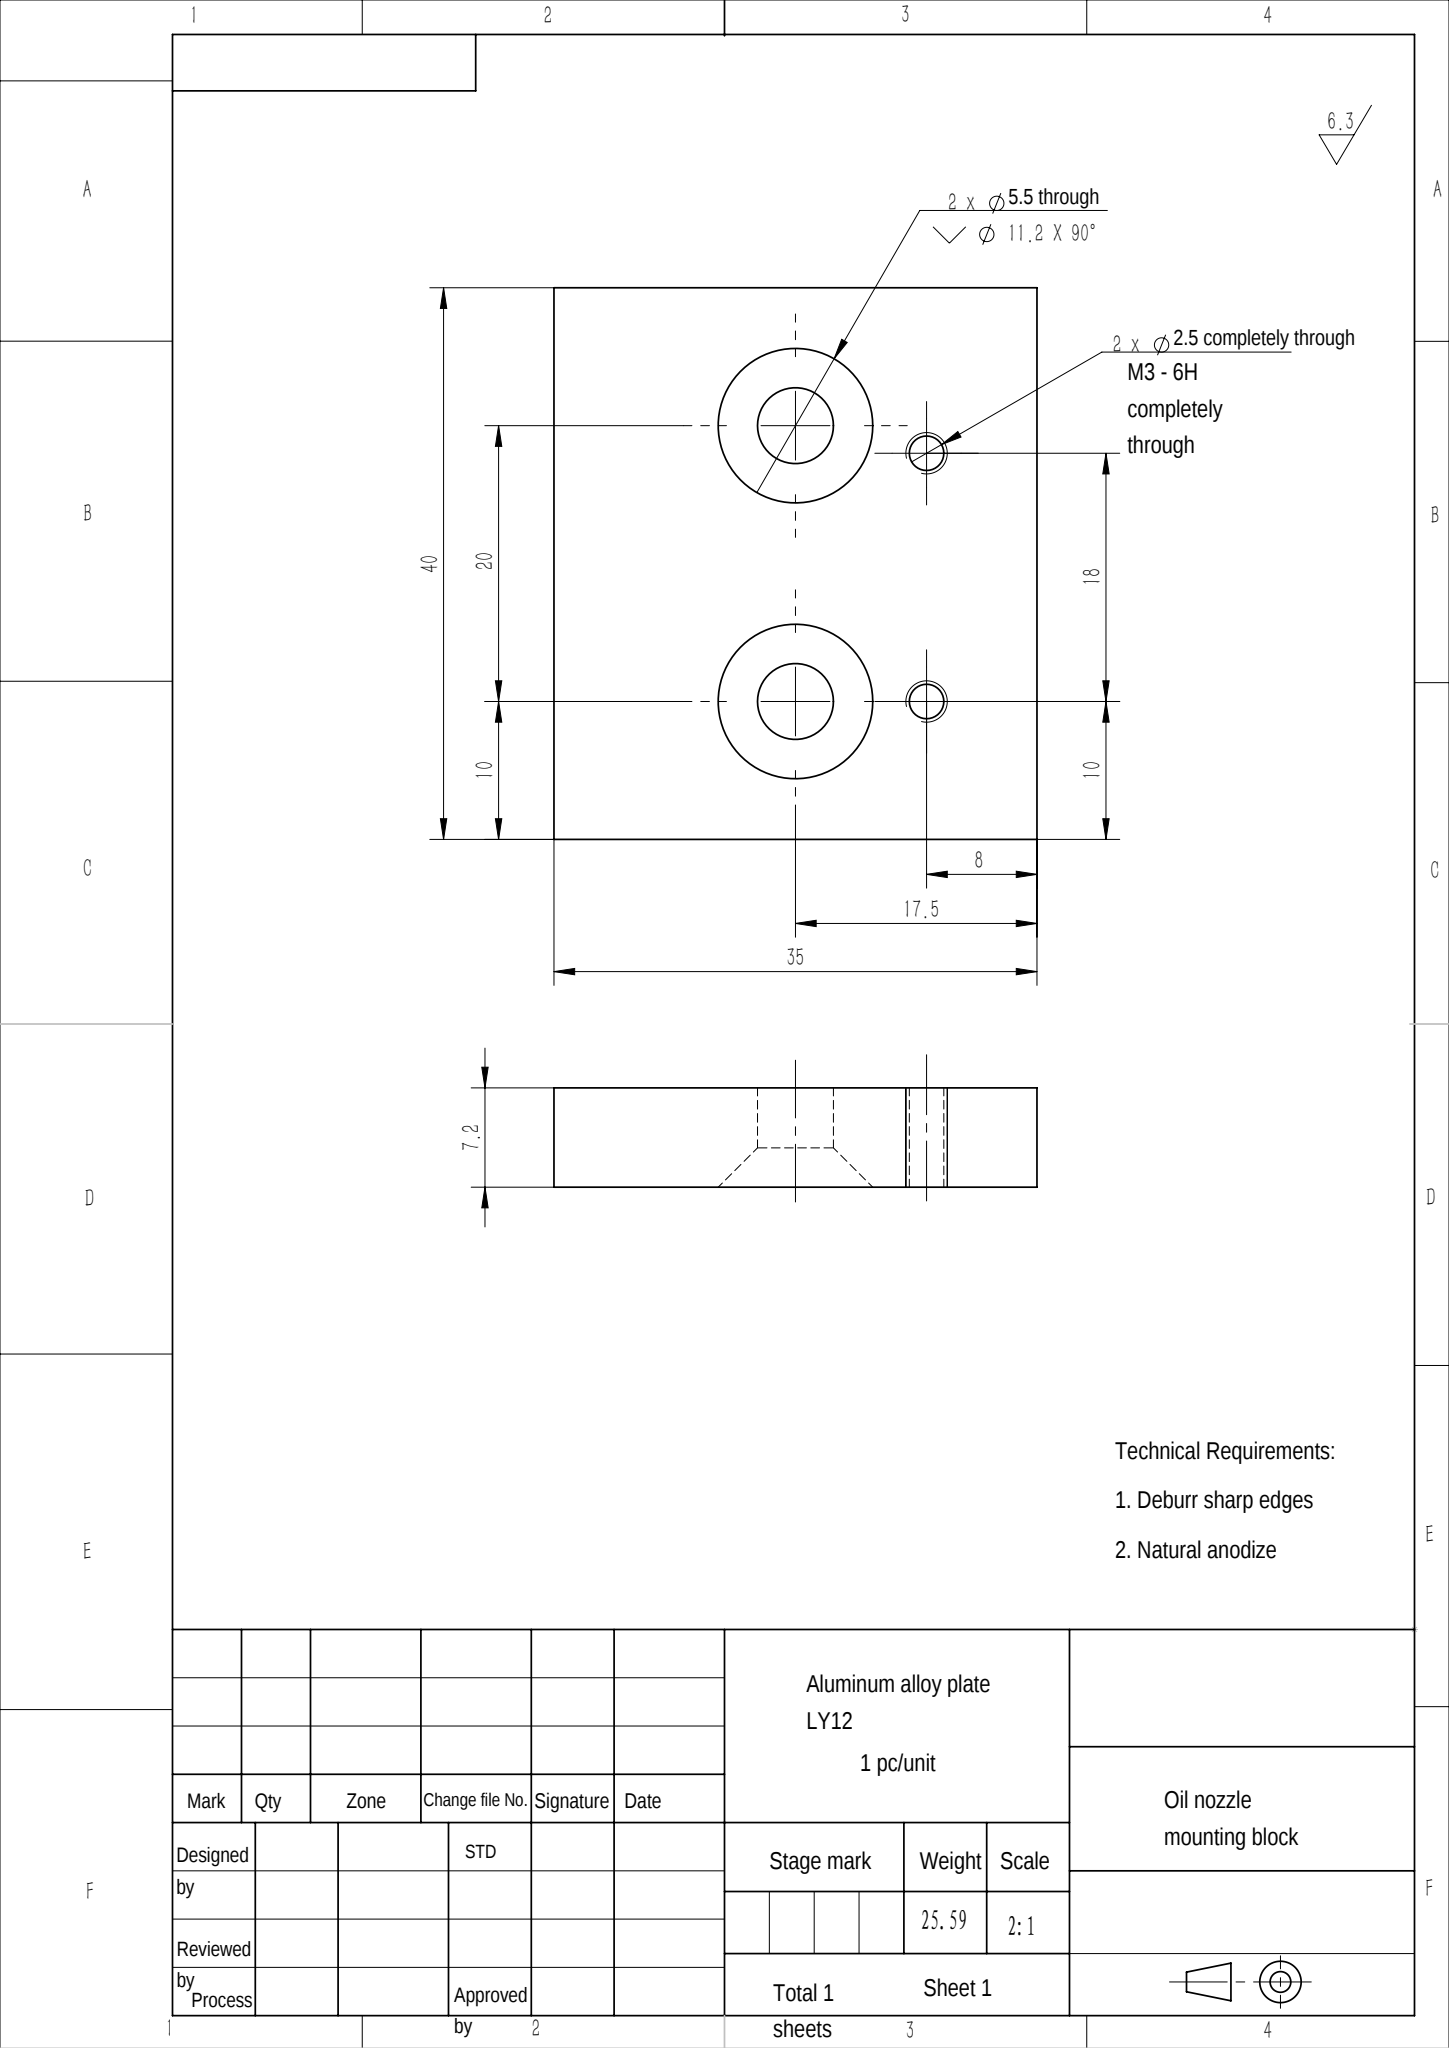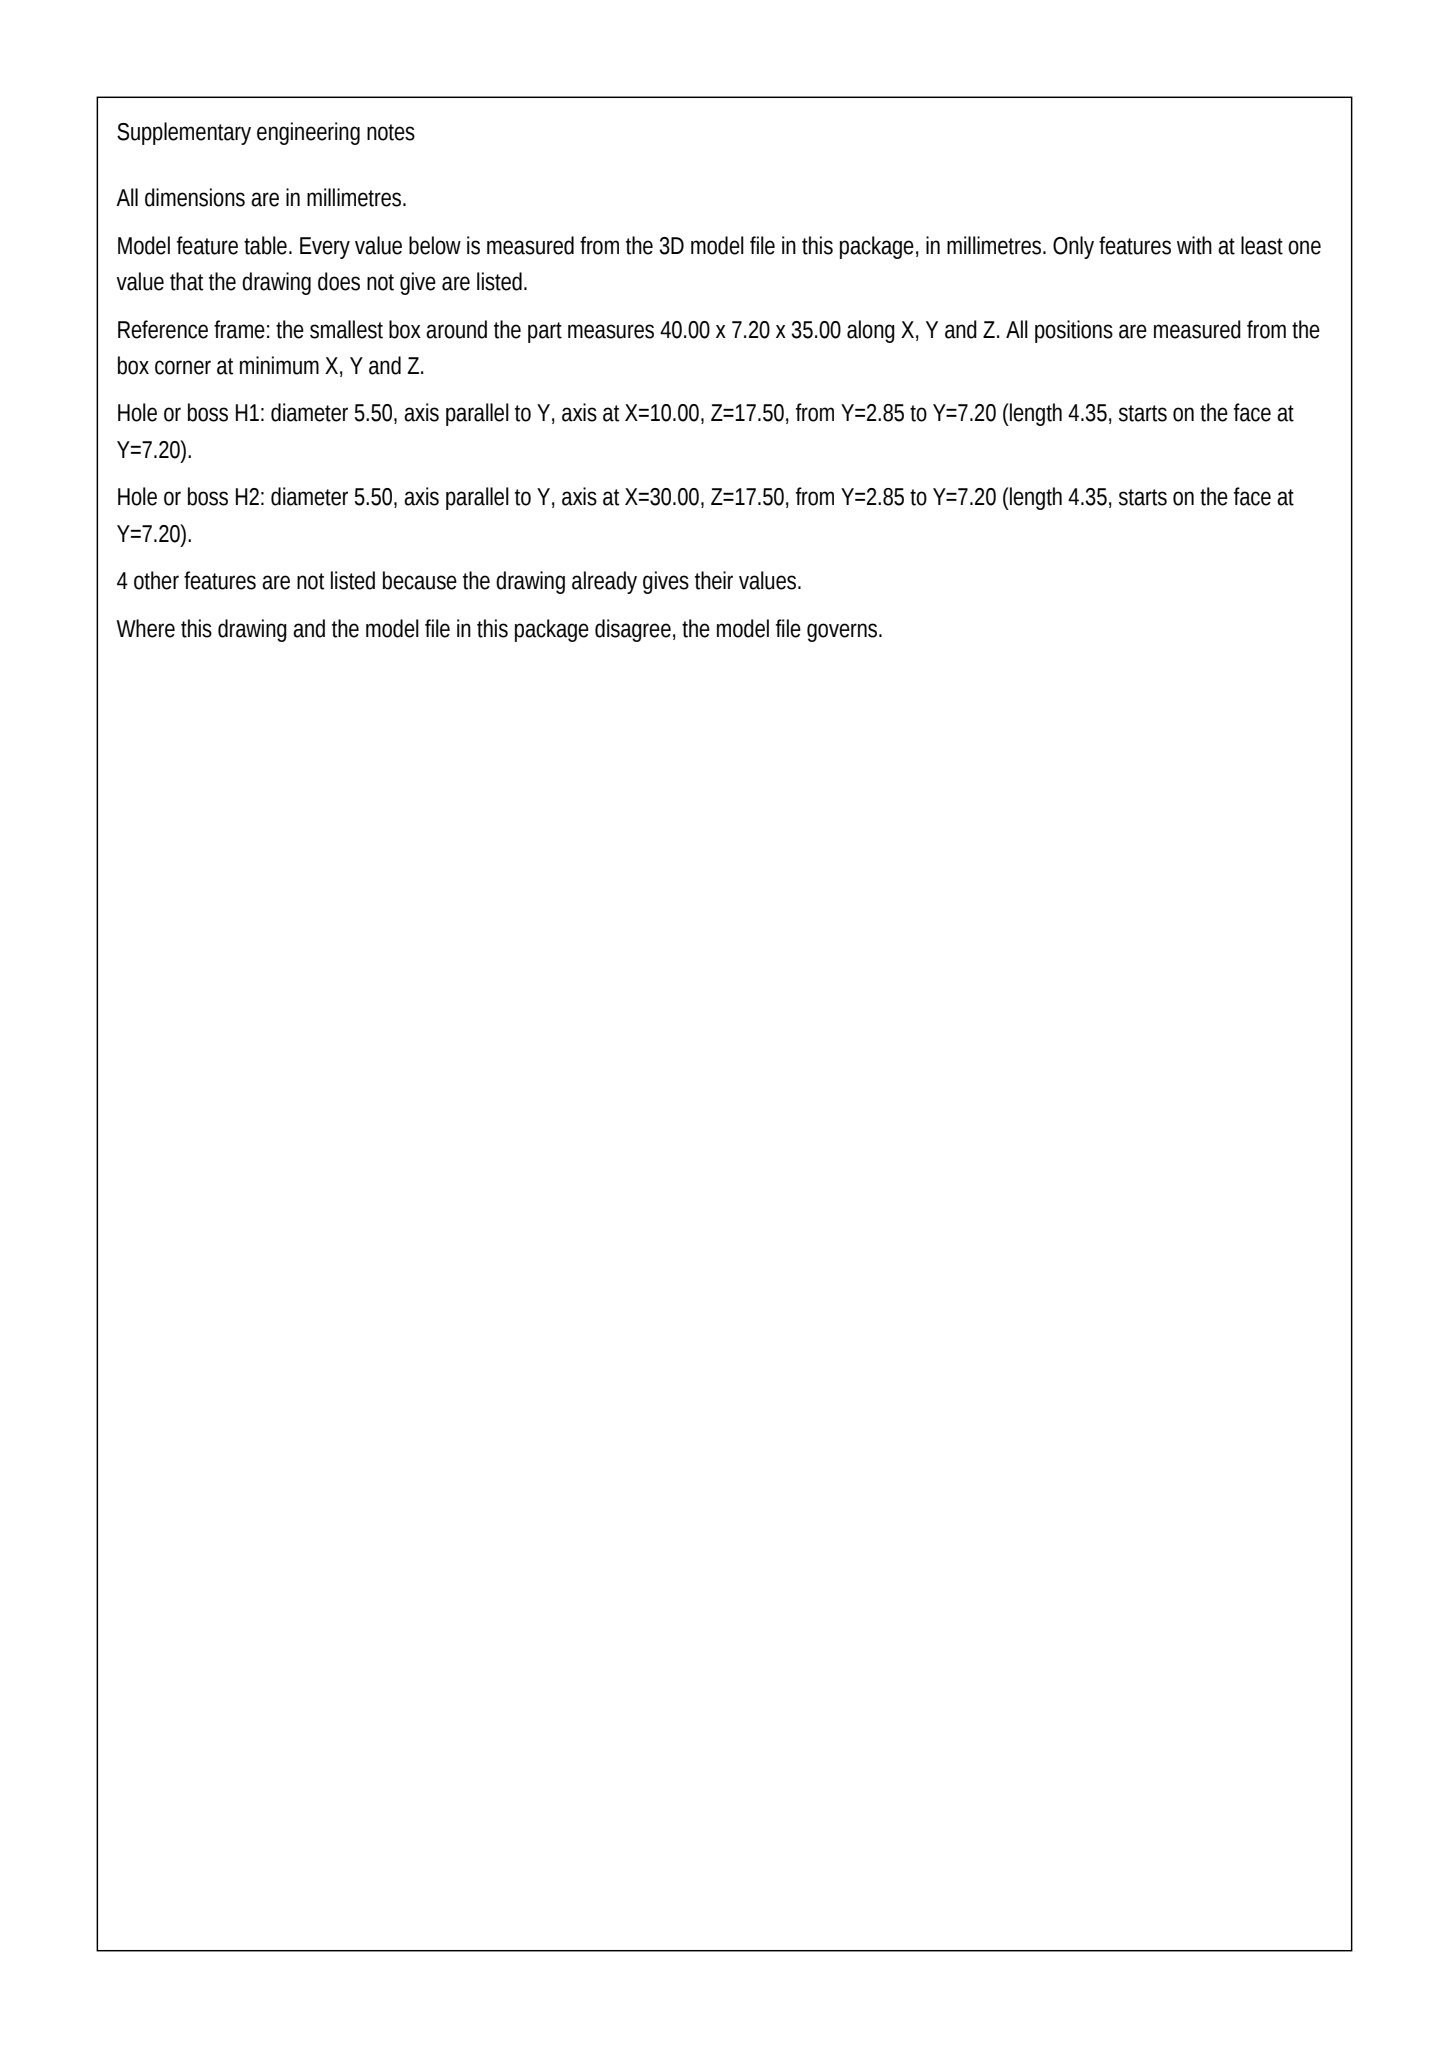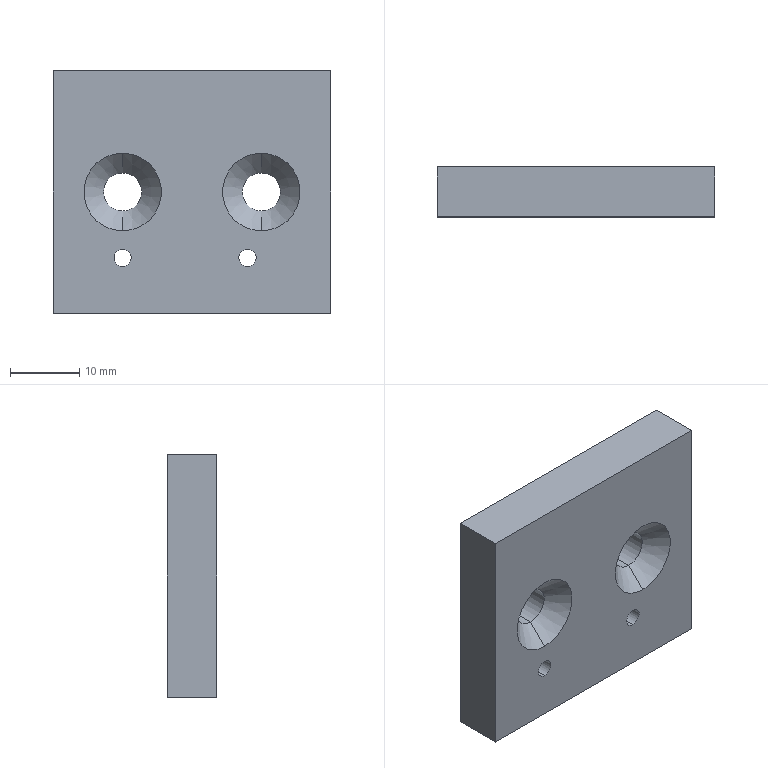Part | SolidWorks | mm | material Aluminum alloy plate LY12 | 1 solid | 18 faces | box 40 x 7.2 x 35 mm | volume 9478 mm3 | cylinder 8 | plane 6 | cone 4 | commonest cylinder face diameters 5.5 x4 2.5 x4
build123d program:
from build123d import *

# Parameters (mm, degrees)
SKETCH1_W                                           = 40
SKETCH1_H                                           = 35
BOSS_EXTRUDE1_DEPTH                                 = 7.2
M3_TAPPED_HOLE1_D                                   = 2.5
TAPERED_COUNTERSUNK_HOLE_FOR_M5_HEXAGON_D           = 5.5
TAPERED_COUNTERSUNK_HOLE_FOR_M5_HEXAGON_CSINK_D     = 11.2
TAPERED_COUNTERSUNK_HOLE_FOR_M5_HEXAGON_CSINK_ANGLE = 90


with BuildPart() as part:
    # Sketch1 → Boss-Extrude1 (new body)
    with BuildSketch(Plane(origin=(0, 0, 0), x_dir=(1, 0, 0), z_dir=(0, 1, 0))):
        Rectangle(SKETCH1_W, SKETCH1_H)
    extrude(amount=BOSS_EXTRUDE1_DEPTH)

    # M3 Tapped Hole1 (through all)
    with Locations(Plane(origin=(0, 0, 0), x_dir=(-1, 0, 0), z_dir=(0, -1, 0))):
        with Locations((10, 9.5), (-8, 9.5)):
            Hole(M3_TAPPED_HOLE1_D / 2)

    # Tapered Countersunk Hole for M5 Hexagon (through all)
    with Locations(Plane(origin=(0, 0, 0), x_dir=(-1, 0, 0), z_dir=(0, -1, 0))):
        with Locations((-10, 0), (10, 0)):
            CounterSinkHole(TAPERED_COUNTERSUNK_HOLE_FOR_M5_HEXAGON_D / 2, TAPERED_COUNTERSUNK_HOLE_FOR_M5_HEXAGON_CSINK_D / 2, counter_sink_angle=TAPERED_COUNTERSUNK_HOLE_FOR_M5_HEXAGON_CSINK_ANGLE)


solid = part.part
STEP:
#1=CARTESIAN_POINT('',(10.,2.85,2.75));
#2=VERTEX_POINT('',#1);
#3=CARTESIAN_POINT('',(10.,2.85,-2.75));
#4=VERTEX_POINT('',#3);
#5=CARTESIAN_POINT('',(10.,2.85,-0.));
#6=DIRECTION('',(0.,-1.,0.));
#7=DIRECTION('',(0.,0.,-1.));
#8=AXIS2_PLACEMENT_3D('',#5,#6,#7);
#9=CIRCLE('',#8,2.75);
#10=EDGE_CURVE('',#2,#4,#9,.T.);
#11=ORIENTED_EDGE('',*,*,#10,.F.);
#12=CARTESIAN_POINT('',(10.,-0.,5.6));
#13=VERTEX_POINT('',#12);
#14=CARTESIAN_POINT('',(10.,-0.,5.6));
#15=DIRECTION('',(0.,-0.7071,0.7071));
#16=VECTOR('',#15,1000.);
#17=LINE('',#14,#16);
#18=EDGE_CURVE('',#2,#13,#17,.T.);
#19=ORIENTED_EDGE('',*,*,#18,.T.);
#20=CARTESIAN_POINT('',(10.,-0.,-5.6));
#21=VERTEX_POINT('',#20);
#22=CARTESIAN_POINT('',(10.,-0.,-0.));
#23=DIRECTION('',(0.,-1.,0.));
#24=DIRECTION('',(0.,0.,-1.));
#25=AXIS2_PLACEMENT_3D('',#22,#23,#24);
#26=CIRCLE('',#25,5.6);
#27=EDGE_CURVE('',#13,#21,#26,.T.);
#28=ORIENTED_EDGE('',*,*,#27,.T.);
#29=CARTESIAN_POINT('',(10.,-0.,-5.6));
#30=DIRECTION('',(0.,-0.7071,-0.7071));
#31=VECTOR('',#30,1000.);
#32=LINE('',#29,#31);
#33=EDGE_CURVE('',#4,#21,#32,.T.);
#34=ORIENTED_EDGE('',*,*,#33,.F.);
#35=EDGE_LOOP('',(#11,#19,#28,#34));
#36=FACE_OUTER_BOUND('',#35,.T.);
#37=CARTESIAN_POINT('',(10.,-0.,-0.));
#38=DIRECTION('',(0.,-1.,0.));
#39=DIRECTION('',(0.,0.,-1.));
#40=AXIS2_PLACEMENT_3D('',#37,#38,#39);
#41=CONICAL_SURFACE('',#40,5.6,0.7854);
#42=ADVANCED_FACE('',(#36),#41,.F.);
#43=CARTESIAN_POINT('',(10.,7.2,-2.75));
#44=VERTEX_POINT('',#43);
#45=CARTESIAN_POINT('',(10.,7.2,2.75));
#46=VERTEX_POINT('',#45);
#47=CARTESIAN_POINT('',(10.,7.2,-0.));
#48=DIRECTION('',(0.,1.,0.));
#49=DIRECTION('',(0.,0.,1.));
#50=AXIS2_PLACEMENT_3D('',#47,#48,#49);
#51=CIRCLE('',#50,2.75);
#52=EDGE_CURVE('',#44,#46,#51,.T.);
#53=ORIENTED_EDGE('',*,*,#52,.T.);
#54=CARTESIAN_POINT('',(10.,0.,2.75));
#55=DIRECTION('',(0.,-1.,0.));
#56=VECTOR('',#55,1000.);
#57=LINE('',#54,#56);
#58=EDGE_CURVE('',#46,#2,#57,.T.);
#59=ORIENTED_EDGE('',*,*,#58,.T.);
#60=ORIENTED_EDGE('',*,*,#10,.T.);
#61=CARTESIAN_POINT('',(10.,0.,-2.75));
#62=DIRECTION('',(0.,-1.,0.));
#63=VECTOR('',#62,1000.);
#64=LINE('',#61,#63);
#65=EDGE_CURVE('',#44,#4,#64,.T.);
#66=ORIENTED_EDGE('',*,*,#65,.F.);
#67=EDGE_LOOP('',(#53,#59,#60,#66));
#68=FACE_OUTER_BOUND('',#67,.T.);
#69=CARTESIAN_POINT('',(10.,0.,-0.));
#70=DIRECTION('',(0.,-1.,0.));
#71=DIRECTION('',(0.,0.,-1.));
#72=AXIS2_PLACEMENT_3D('',#69,#70,#71);
#73=CYLINDRICAL_SURFACE('',#72,2.75);
#74=ADVANCED_FACE('',(#68),#73,.F.);
#75=CARTESIAN_POINT('',(-10.,2.85,2.75));
#76=VERTEX_POINT('',#75);
#77=CARTESIAN_POINT('',(-10.,2.85,-2.75));
#78=VERTEX_POINT('',#77);
#79=CARTESIAN_POINT('',(-10.,2.85,-0.));
#80=DIRECTION('',(0.,-1.,0.));
#81=DIRECTION('',(0.,0.,-1.));
#82=AXIS2_PLACEMENT_3D('',#79,#80,#81);
#83=CIRCLE('',#82,2.75);
#84=EDGE_CURVE('',#76,#78,#83,.T.);
#85=ORIENTED_EDGE('',*,*,#84,.F.);
#86=CARTESIAN_POINT('',(-10.,-0.,5.6));
#87=VERTEX_POINT('',#86);
#88=CARTESIAN_POINT('',(-10.,-0.,5.6));
#89=DIRECTION('',(0.,-0.7071,0.7071));
#90=VECTOR('',#89,1000.);
#91=LINE('',#88,#90);
#92=EDGE_CURVE('',#76,#87,#91,.T.);
#93=ORIENTED_EDGE('',*,*,#92,.T.);
#94=CARTESIAN_POINT('',(-10.,-0.,-5.6));
#95=VERTEX_POINT('',#94);
#96=CARTESIAN_POINT('',(-10.,-0.,-0.));
#97=DIRECTION('',(0.,-1.,0.));
#98=DIRECTION('',(0.,0.,-1.));
#99=AXIS2_PLACEMENT_3D('',#96,#97,#98);
#100=CIRCLE('',#99,5.6);
#101=EDGE_CURVE('',#87,#95,#100,.T.);
#102=ORIENTED_EDGE('',*,*,#101,.T.);
#103=CARTESIAN_POINT('',(-10.,-0.,-5.6));
#104=DIRECTION('',(0.,-0.7071,-0.7071));
#105=VECTOR('',#104,1000.);
#106=LINE('',#103,#105);
#107=EDGE_CURVE('',#78,#95,#106,.T.);
#108=ORIENTED_EDGE('',*,*,#107,.F.);
#109=EDGE_LOOP('',(#85,#93,#102,#108));
#110=FACE_OUTER_BOUND('',#109,.T.);
#111=CARTESIAN_POINT('',(-10.,-0.,-0.));
#112=DIRECTION('',(0.,-1.,0.));
#113=DIRECTION('',(0.,0.,-1.));
#114=AXIS2_PLACEMENT_3D('',#111,#112,#113);
#115=CONICAL_SURFACE('',#114,5.6,0.7854);
#116=ADVANCED_FACE('',(#110),#115,.F.);
#117=CARTESIAN_POINT('',(-10.,7.2,-2.75));
#118=VERTEX_POINT('',#117);
#119=CARTESIAN_POINT('',(-10.,7.2,2.75));
#120=VERTEX_POINT('',#119);
#121=CARTESIAN_POINT('',(-10.,7.2,-0.));
#122=DIRECTION('',(0.,1.,0.));
#123=DIRECTION('',(0.,0.,1.));
#124=AXIS2_PLACEMENT_3D('',#121,#122,#123);
#125=CIRCLE('',#124,2.75);
#126=EDGE_CURVE('',#118,#120,#125,.T.);
#127=ORIENTED_EDGE('',*,*,#126,.T.);
#128=CARTESIAN_POINT('',(-10.,0.,2.75));
#129=DIRECTION('',(0.,-1.,0.));
#130=VECTOR('',#129,1000.);
#131=LINE('',#128,#130);
#132=EDGE_CURVE('',#120,#76,#131,.T.);
#133=ORIENTED_EDGE('',*,*,#132,.T.);
#134=ORIENTED_EDGE('',*,*,#84,.T.);
#135=CARTESIAN_POINT('',(-10.,0.,-2.75));
#136=DIRECTION('',(0.,-1.,0.));
#137=VECTOR('',#136,1000.);
#138=LINE('',#135,#137);
#139=EDGE_CURVE('',#118,#78,#138,.T.);
#140=ORIENTED_EDGE('',*,*,#139,.F.);
#141=EDGE_LOOP('',(#127,#133,#134,#140));
#142=FACE_OUTER_BOUND('',#141,.T.);
#143=CARTESIAN_POINT('',(-10.,0.,-0.));
#144=DIRECTION('',(0.,-1.,0.));
#145=DIRECTION('',(0.,0.,-1.));
#146=AXIS2_PLACEMENT_3D('',#143,#144,#145);
#147=CYLINDRICAL_SURFACE('',#146,2.75);
#148=ADVANCED_FACE('',(#142),#147,.F.);
#149=CARTESIAN_POINT('',(-10.,7.2,-8.25));
#150=VERTEX_POINT('',#149);
#151=CARTESIAN_POINT('',(-10.,7.2,-10.75));
#152=VERTEX_POINT('',#151);
#153=CARTESIAN_POINT('',(-10.,7.2,-9.5));
#154=DIRECTION('',(0.,-1.,0.));
#155=DIRECTION('',(0.,0.,-1.));
#156=AXIS2_PLACEMENT_3D('',#153,#154,#155);
#157=CIRCLE('',#156,1.25);
#158=EDGE_CURVE('',#150,#152,#157,.T.);
#159=ORIENTED_EDGE('',*,*,#158,.F.);
#160=CARTESIAN_POINT('',(-10.,0.,-8.25));
#161=VERTEX_POINT('',#160);
#162=CARTESIAN_POINT('',(-10.,0.,-8.25));
#163=DIRECTION('',(0.,-1.,0.));
#164=VECTOR('',#163,1000.);
#165=LINE('',#162,#164);
#166=EDGE_CURVE('',#150,#161,#165,.T.);
#167=ORIENTED_EDGE('',*,*,#166,.T.);
#168=CARTESIAN_POINT('',(-10.,0.,-10.75));
#169=VERTEX_POINT('',#168);
#170=CARTESIAN_POINT('',(-10.,0.,-9.5));
#171=DIRECTION('',(0.,-1.,0.));
#172=DIRECTION('',(0.,0.,-1.));
#173=AXIS2_PLACEMENT_3D('',#170,#171,#172);
#174=CIRCLE('',#173,1.25);
#175=EDGE_CURVE('',#161,#169,#174,.T.);
#176=ORIENTED_EDGE('',*,*,#175,.T.);
#177=CARTESIAN_POINT('',(-10.,0.,-10.75));
#178=DIRECTION('',(0.,-1.,0.));
#179=VECTOR('',#178,1000.);
#180=LINE('',#177,#179);
#181=EDGE_CURVE('',#152,#169,#180,.T.);
#182=ORIENTED_EDGE('',*,*,#181,.F.);
#183=EDGE_LOOP('',(#159,#167,#176,#182));
#184=FACE_OUTER_BOUND('',#183,.T.);
#185=CARTESIAN_POINT('',(-10.,0.,-9.5));
#186=DIRECTION('',(0.,-1.,0.));
#187=DIRECTION('',(0.,0.,-1.));
#188=AXIS2_PLACEMENT_3D('',#185,#186,#187);
#189=CYLINDRICAL_SURFACE('',#188,1.25);
#190=ADVANCED_FACE('',(#184),#189,.F.);
#191=CARTESIAN_POINT('',(8.,7.2,-8.25));
#192=VERTEX_POINT('',#191);
#193=CARTESIAN_POINT('',(8.,7.2,-10.75));
#194=VERTEX_POINT('',#193);
#195=CARTESIAN_POINT('',(8.,7.2,-9.5));
#196=DIRECTION('',(0.,-1.,0.));
#197=DIRECTION('',(0.,0.,-1.));
#198=AXIS2_PLACEMENT_3D('',#195,#196,#197);
#199=CIRCLE('',#198,1.25);
#200=EDGE_CURVE('',#192,#194,#199,.T.);
#201=ORIENTED_EDGE('',*,*,#200,.F.);
#202=CARTESIAN_POINT('',(8.,0.,-8.25));
#203=VERTEX_POINT('',#202);
#204=CARTESIAN_POINT('',(8.,0.,-8.25));
#205=DIRECTION('',(0.,-1.,0.));
#206=VECTOR('',#205,1000.);
#207=LINE('',#204,#206);
#208=EDGE_CURVE('',#192,#203,#207,.T.);
#209=ORIENTED_EDGE('',*,*,#208,.T.);
#210=CARTESIAN_POINT('',(8.,0.,-10.75));
#211=VERTEX_POINT('',#210);
#212=CARTESIAN_POINT('',(8.,0.,-9.5));
#213=DIRECTION('',(0.,-1.,0.));
#214=DIRECTION('',(0.,0.,-1.));
#215=AXIS2_PLACEMENT_3D('',#212,#213,#214);
#216=CIRCLE('',#215,1.25);
#217=EDGE_CURVE('',#203,#211,#216,.T.);
#218=ORIENTED_EDGE('',*,*,#217,.T.);
#219=CARTESIAN_POINT('',(8.,0.,-10.75));
#220=DIRECTION('',(0.,-1.,0.));
#221=VECTOR('',#220,1000.);
#222=LINE('',#219,#221);
#223=EDGE_CURVE('',#194,#211,#222,.T.);
#224=ORIENTED_EDGE('',*,*,#223,.F.);
#225=EDGE_LOOP('',(#201,#209,#218,#224));
#226=FACE_OUTER_BOUND('',#225,.T.);
#227=CARTESIAN_POINT('',(8.,0.,-9.5));
#228=DIRECTION('',(0.,-1.,0.));
#229=DIRECTION('',(0.,0.,-1.));
#230=AXIS2_PLACEMENT_3D('',#227,#228,#229);
#231=CYLINDRICAL_SURFACE('',#230,1.25);
#232=ADVANCED_FACE('',(#226),#231,.F.);
#233=CARTESIAN_POINT('',(-10.,-0.,-0.));
#234=DIRECTION('',(0.,-1.,0.));
#235=DIRECTION('',(0.,0.,-1.));
#236=AXIS2_PLACEMENT_3D('',#233,#234,#235);
#237=CIRCLE('',#236,5.6);
#238=EDGE_CURVE('',#95,#87,#237,.T.);
#239=ORIENTED_EDGE('',*,*,#238,.F.);
#240=ORIENTED_EDGE('',*,*,#101,.F.);
#241=EDGE_LOOP('',(#239,#240));
#242=FACE_BOUND('',#241,.T.);
#243=CARTESIAN_POINT('',(-10.,0.,-9.5));
#244=DIRECTION('',(0.,-1.,0.));
#245=DIRECTION('',(0.,0.,-1.));
#246=AXIS2_PLACEMENT_3D('',#243,#244,#245);
#247=CIRCLE('',#246,1.25);
#248=EDGE_CURVE('',#169,#161,#247,.T.);
#249=ORIENTED_EDGE('',*,*,#248,.F.);
#250=ORIENTED_EDGE('',*,*,#175,.F.);
#251=EDGE_LOOP('',(#249,#250));
#252=FACE_BOUND('',#251,.T.);
#253=CARTESIAN_POINT('',(8.,0.,-9.5));
#254=DIRECTION('',(0.,-1.,0.));
#255=DIRECTION('',(0.,0.,-1.));
#256=AXIS2_PLACEMENT_3D('',#253,#254,#255);
#257=CIRCLE('',#256,1.25);
#258=EDGE_CURVE('',#211,#203,#257,.T.);
#259=ORIENTED_EDGE('',*,*,#258,.F.);
#260=ORIENTED_EDGE('',*,*,#217,.F.);
#261=EDGE_LOOP('',(#259,#260));
#262=FACE_BOUND('',#261,.T.);
#263=CARTESIAN_POINT('',(20.,0.,17.5));
#264=VERTEX_POINT('',#263);
#265=CARTESIAN_POINT('',(20.,0.,-17.5));
#266=VERTEX_POINT('',#265);
#267=CARTESIAN_POINT('',(20.,0.,-17.5));
#268=DIRECTION('',(0.,0.,-1.));
#269=VECTOR('',#268,1000.);
#270=LINE('',#267,#269);
#271=EDGE_CURVE('',#264,#266,#270,.T.);
#272=ORIENTED_EDGE('',*,*,#271,.F.);
#273=CARTESIAN_POINT('',(-20.,0.,17.5));
#274=VERTEX_POINT('',#273);
#275=CARTESIAN_POINT('',(-20.,0.,17.5));
#276=DIRECTION('',(1.,0.,0.));
#277=VECTOR('',#276,1000.);
#278=LINE('',#275,#277);
#279=EDGE_CURVE('',#274,#264,#278,.T.);
#280=ORIENTED_EDGE('',*,*,#279,.F.);
#281=CARTESIAN_POINT('',(-20.,0.,-17.5));
#282=VERTEX_POINT('',#281);
#283=CARTESIAN_POINT('',(-20.,0.,-17.5));
#284=DIRECTION('',(0.,0.,1.));
#285=VECTOR('',#284,1000.);
#286=LINE('',#283,#285);
#287=EDGE_CURVE('',#282,#274,#286,.T.);
#288=ORIENTED_EDGE('',*,*,#287,.F.);
#289=CARTESIAN_POINT('',(-20.,0.,-17.5));
#290=DIRECTION('',(-1.,0.,-0.));
#291=VECTOR('',#290,1000.);
#292=LINE('',#289,#291);
#293=EDGE_CURVE('',#266,#282,#292,.T.);
#294=ORIENTED_EDGE('',*,*,#293,.F.);
#295=EDGE_LOOP('',(#272,#280,#288,#294));
#296=FACE_OUTER_BOUND('',#295,.T.);
#297=CARTESIAN_POINT('',(10.,-0.,-0.));
#298=DIRECTION('',(0.,-1.,0.));
#299=DIRECTION('',(0.,0.,-1.));
#300=AXIS2_PLACEMENT_3D('',#297,#298,#299);
#301=CIRCLE('',#300,5.6);
#302=EDGE_CURVE('',#21,#13,#301,.T.);
#303=ORIENTED_EDGE('',*,*,#302,.F.);
#304=ORIENTED_EDGE('',*,*,#27,.F.);
#305=EDGE_LOOP('',(#303,#304));
#306=FACE_BOUND('',#305,.T.);
#307=CARTESIAN_POINT('',(0.,0.,0.));
#308=DIRECTION('',(0.,1.,0.));
#309=DIRECTION('',(0.,0.,1.));
#310=AXIS2_PLACEMENT_3D('',#307,#308,#309);
#311=PLANE('',#310);
#312=ADVANCED_FACE('',(#242,#252,#262,#296,#306),#311,.F.);
#313=ORIENTED_EDGE('',*,*,#271,.T.);
#314=CARTESIAN_POINT('',(20.,7.2,-17.5));
#315=VERTEX_POINT('',#314);
#316=CARTESIAN_POINT('',(20.,7.2,-17.5));
#317=DIRECTION('',(0.,-1.,0.));
#318=VECTOR('',#317,1000.);
#319=LINE('',#316,#318);
#320=EDGE_CURVE('',#315,#266,#319,.T.);
#321=ORIENTED_EDGE('',*,*,#320,.F.);
#322=CARTESIAN_POINT('',(20.,7.2,17.5));
#323=VERTEX_POINT('',#322);
#324=CARTESIAN_POINT('',(20.,7.2,-17.5));
#325=DIRECTION('',(0.,0.,-1.));
#326=VECTOR('',#325,1000.);
#327=LINE('',#324,#326);
#328=EDGE_CURVE('',#323,#315,#327,.T.);
#329=ORIENTED_EDGE('',*,*,#328,.F.);
#330=CARTESIAN_POINT('',(20.,7.2,17.5));
#331=DIRECTION('',(0.,-1.,0.));
#332=VECTOR('',#331,1000.);
#333=LINE('',#330,#332);
#334=EDGE_CURVE('',#323,#264,#333,.T.);
#335=ORIENTED_EDGE('',*,*,#334,.T.);
#336=EDGE_LOOP('',(#313,#321,#329,#335));
#337=FACE_OUTER_BOUND('',#336,.T.);
#338=CARTESIAN_POINT('',(20.,7.2,-17.5));
#339=DIRECTION('',(-1.,0.,-0.));
#340=DIRECTION('',(-0.,0.,1.));
#341=AXIS2_PLACEMENT_3D('',#338,#339,#340);
#342=PLANE('',#341);
#343=ADVANCED_FACE('',(#337),#342,.F.);
#344=ORIENTED_EDGE('',*,*,#293,.T.);
#345=CARTESIAN_POINT('',(-20.,7.2,-17.5));
#346=VERTEX_POINT('',#345);
#347=CARTESIAN_POINT('',(-20.,7.2,-17.5));
#348=DIRECTION('',(0.,-1.,0.));
#349=VECTOR('',#348,1000.);
#350=LINE('',#347,#349);
#351=EDGE_CURVE('',#346,#282,#350,.T.);
#352=ORIENTED_EDGE('',*,*,#351,.F.);
#353=CARTESIAN_POINT('',(-20.,7.2,-17.5));
#354=DIRECTION('',(-1.,0.,-0.));
#355=VECTOR('',#354,1000.);
#356=LINE('',#353,#355);
#357=EDGE_CURVE('',#315,#346,#356,.T.);
#358=ORIENTED_EDGE('',*,*,#357,.F.);
#359=ORIENTED_EDGE('',*,*,#320,.T.);
#360=EDGE_LOOP('',(#344,#352,#358,#359));
#361=FACE_OUTER_BOUND('',#360,.T.);
#362=CARTESIAN_POINT('',(-20.,7.2,-17.5));
#363=DIRECTION('',(-0.,0.,1.));
#364=DIRECTION('',(1.,0.,0.));
#365=AXIS2_PLACEMENT_3D('',#362,#363,#364);
#366=PLANE('',#365);
#367=ADVANCED_FACE('',(#361),#366,.F.);
#368=ORIENTED_EDGE('',*,*,#287,.T.);
#369=CARTESIAN_POINT('',(-20.,7.2,17.5));
#370=VERTEX_POINT('',#369);
#371=CARTESIAN_POINT('',(-20.,7.2,17.5));
#372=DIRECTION('',(0.,-1.,0.));
#373=VECTOR('',#372,1000.);
#374=LINE('',#371,#373);
#375=EDGE_CURVE('',#370,#274,#374,.T.);
#376=ORIENTED_EDGE('',*,*,#375,.F.);
#377=CARTESIAN_POINT('',(-20.,7.2,-17.5));
#378=DIRECTION('',(0.,0.,1.));
#379=VECTOR('',#378,1000.);
#380=LINE('',#377,#379);
#381=EDGE_CURVE('',#346,#370,#380,.T.);
#382=ORIENTED_EDGE('',*,*,#381,.F.);
#383=ORIENTED_EDGE('',*,*,#351,.T.);
#384=EDGE_LOOP('',(#368,#376,#382,#383));
#385=FACE_OUTER_BOUND('',#384,.T.);
#386=CARTESIAN_POINT('',(-20.,7.2,-17.5));
#387=DIRECTION('',(1.,0.,0.));
#388=DIRECTION('',(0.,0.,-1.));
#389=AXIS2_PLACEMENT_3D('',#386,#387,#388);
#390=PLANE('',#389);
#391=ADVANCED_FACE('',(#385),#390,.F.);
#392=ORIENTED_EDGE('',*,*,#279,.T.);
#393=ORIENTED_EDGE('',*,*,#334,.F.);
#394=CARTESIAN_POINT('',(-20.,7.2,17.5));
#395=DIRECTION('',(1.,0.,0.));
#396=VECTOR('',#395,1000.);
#397=LINE('',#394,#396);
#398=EDGE_CURVE('',#370,#323,#397,.T.);
#399=ORIENTED_EDGE('',*,*,#398,.F.);
#400=ORIENTED_EDGE('',*,*,#375,.T.);
#401=EDGE_LOOP('',(#392,#393,#399,#400));
#402=FACE_OUTER_BOUND('',#401,.T.);
#403=CARTESIAN_POINT('',(-20.,7.2,17.5));
#404=DIRECTION('',(0.,0.,-1.));
#405=DIRECTION('',(-1.,0.,0.));
#406=AXIS2_PLACEMENT_3D('',#403,#404,#405);
#407=PLANE('',#406);
#408=ADVANCED_FACE('',(#402),#407,.F.);
#409=ORIENTED_EDGE('',*,*,#52,.F.);
#410=CARTESIAN_POINT('',(10.,7.2,-0.));
#411=DIRECTION('',(0.,1.,0.));
#412=DIRECTION('',(0.,0.,1.));
#413=AXIS2_PLACEMENT_3D('',#410,#411,#412);
#414=CIRCLE('',#413,2.75);
#415=EDGE_CURVE('',#46,#44,#414,.T.);
#416=ORIENTED_EDGE('',*,*,#415,.F.);
#417=EDGE_LOOP('',(#409,#416));
#418=FACE_BOUND('',#417,.T.);
#419=ORIENTED_EDGE('',*,*,#126,.F.);
#420=CARTESIAN_POINT('',(-10.,7.2,-0.));
#421=DIRECTION('',(0.,1.,0.));
#422=DIRECTION('',(0.,0.,1.));
#423=AXIS2_PLACEMENT_3D('',#420,#421,#422);
#424=CIRCLE('',#423,2.75);
#425=EDGE_CURVE('',#120,#118,#424,.T.);
#426=ORIENTED_EDGE('',*,*,#425,.F.);
#427=EDGE_LOOP('',(#419,#426));
#428=FACE_BOUND('',#427,.T.);
#429=CARTESIAN_POINT('',(-10.,7.2,-9.5));
#430=DIRECTION('',(0.,-1.,0.));
#431=DIRECTION('',(0.,0.,-1.));
#432=AXIS2_PLACEMENT_3D('',#429,#430,#431);
#433=CIRCLE('',#432,1.25);
#434=EDGE_CURVE('',#152,#150,#433,.T.);
#435=ORIENTED_EDGE('',*,*,#434,.T.);
#436=ORIENTED_EDGE('',*,*,#158,.T.);
#437=EDGE_LOOP('',(#435,#436));
#438=FACE_BOUND('',#437,.T.);
#439=CARTESIAN_POINT('',(8.,7.2,-9.5));
#440=DIRECTION('',(0.,-1.,0.));
#441=DIRECTION('',(0.,0.,-1.));
#442=AXIS2_PLACEMENT_3D('',#439,#440,#441);
#443=CIRCLE('',#442,1.25);
#444=EDGE_CURVE('',#194,#192,#443,.T.);
#445=ORIENTED_EDGE('',*,*,#444,.T.);
#446=ORIENTED_EDGE('',*,*,#200,.T.);
#447=EDGE_LOOP('',(#445,#446));
#448=FACE_BOUND('',#447,.T.);
#449=ORIENTED_EDGE('',*,*,#328,.T.);
#450=ORIENTED_EDGE('',*,*,#357,.T.);
#451=ORIENTED_EDGE('',*,*,#381,.T.);
#452=ORIENTED_EDGE('',*,*,#398,.T.);
#453=EDGE_LOOP('',(#449,#450,#451,#452));
#454=FACE_OUTER_BOUND('',#453,.T.);
#455=CARTESIAN_POINT('',(0.,7.2,0.));
#456=DIRECTION('',(0.,1.,0.));
#457=DIRECTION('',(0.,0.,1.));
#458=AXIS2_PLACEMENT_3D('',#455,#456,#457);
#459=PLANE('',#458);
#460=ADVANCED_FACE('',(#418,#428,#438,#448,#454),#459,.T.);
#461=ORIENTED_EDGE('',*,*,#208,.F.);
#462=ORIENTED_EDGE('',*,*,#444,.F.);
#463=ORIENTED_EDGE('',*,*,#223,.T.);
#464=ORIENTED_EDGE('',*,*,#258,.T.);
#465=EDGE_LOOP('',(#461,#462,#463,#464));
#466=FACE_OUTER_BOUND('',#465,.T.);
#467=CARTESIAN_POINT('',(8.,0.,-9.5));
#468=DIRECTION('',(0.,-1.,0.));
#469=DIRECTION('',(0.,0.,-1.));
#470=AXIS2_PLACEMENT_3D('',#467,#468,#469);
#471=CYLINDRICAL_SURFACE('',#470,1.25);
#472=ADVANCED_FACE('',(#466),#471,.F.);
#473=ORIENTED_EDGE('',*,*,#166,.F.);
#474=ORIENTED_EDGE('',*,*,#434,.F.);
#475=ORIENTED_EDGE('',*,*,#181,.T.);
#476=ORIENTED_EDGE('',*,*,#248,.T.);
#477=EDGE_LOOP('',(#473,#474,#475,#476));
#478=FACE_OUTER_BOUND('',#477,.T.);
#479=CARTESIAN_POINT('',(-10.,0.,-9.5));
#480=DIRECTION('',(0.,-1.,0.));
#481=DIRECTION('',(0.,0.,-1.));
#482=AXIS2_PLACEMENT_3D('',#479,#480,#481);
#483=CYLINDRICAL_SURFACE('',#482,1.25);
#484=ADVANCED_FACE('',(#478),#483,.F.);
#485=ORIENTED_EDGE('',*,*,#132,.F.);
#486=ORIENTED_EDGE('',*,*,#425,.T.);
#487=ORIENTED_EDGE('',*,*,#139,.T.);
#488=CARTESIAN_POINT('',(-10.,2.85,-0.));
#489=DIRECTION('',(0.,-1.,0.));
#490=DIRECTION('',(0.,0.,-1.));
#491=AXIS2_PLACEMENT_3D('',#488,#489,#490);
#492=CIRCLE('',#491,2.75);
#493=EDGE_CURVE('',#78,#76,#492,.T.);
#494=ORIENTED_EDGE('',*,*,#493,.T.);
#495=EDGE_LOOP('',(#485,#486,#487,#494));
#496=FACE_OUTER_BOUND('',#495,.T.);
#497=CARTESIAN_POINT('',(-10.,0.,-0.));
#498=DIRECTION('',(0.,-1.,0.));
#499=DIRECTION('',(0.,0.,-1.));
#500=AXIS2_PLACEMENT_3D('',#497,#498,#499);
#501=CYLINDRICAL_SURFACE('',#500,2.75);
#502=ADVANCED_FACE('',(#496),#501,.F.);
#503=ORIENTED_EDGE('',*,*,#92,.F.);
#504=ORIENTED_EDGE('',*,*,#493,.F.);
#505=ORIENTED_EDGE('',*,*,#107,.T.);
#506=ORIENTED_EDGE('',*,*,#238,.T.);
#507=EDGE_LOOP('',(#503,#504,#505,#506));
#508=FACE_OUTER_BOUND('',#507,.T.);
#509=CARTESIAN_POINT('',(-10.,-0.,-0.));
#510=DIRECTION('',(0.,-1.,0.));
#511=DIRECTION('',(0.,0.,-1.));
#512=AXIS2_PLACEMENT_3D('',#509,#510,#511);
#513=CONICAL_SURFACE('',#512,5.6,0.7854);
#514=ADVANCED_FACE('',(#508),#513,.F.);
#515=ORIENTED_EDGE('',*,*,#58,.F.);
#516=ORIENTED_EDGE('',*,*,#415,.T.);
#517=ORIENTED_EDGE('',*,*,#65,.T.);
#518=CARTESIAN_POINT('',(10.,2.85,-0.));
#519=DIRECTION('',(0.,-1.,0.));
#520=DIRECTION('',(0.,0.,-1.));
#521=AXIS2_PLACEMENT_3D('',#518,#519,#520);
#522=CIRCLE('',#521,2.75);
#523=EDGE_CURVE('',#4,#2,#522,.T.);
#524=ORIENTED_EDGE('',*,*,#523,.T.);
#525=EDGE_LOOP('',(#515,#516,#517,#524));
#526=FACE_OUTER_BOUND('',#525,.T.);
#527=CARTESIAN_POINT('',(10.,0.,-0.));
#528=DIRECTION('',(0.,-1.,0.));
#529=DIRECTION('',(0.,0.,-1.));
#530=AXIS2_PLACEMENT_3D('',#527,#528,#529);
#531=CYLINDRICAL_SURFACE('',#530,2.75);
#532=ADVANCED_FACE('',(#526),#531,.F.);
#533=ORIENTED_EDGE('',*,*,#18,.F.);
#534=ORIENTED_EDGE('',*,*,#523,.F.);
#535=ORIENTED_EDGE('',*,*,#33,.T.);
#536=ORIENTED_EDGE('',*,*,#302,.T.);
#537=EDGE_LOOP('',(#533,#534,#535,#536));
#538=FACE_OUTER_BOUND('',#537,.T.);
#539=CARTESIAN_POINT('',(10.,-0.,-0.));
#540=DIRECTION('',(0.,-1.,0.));
#541=DIRECTION('',(0.,0.,-1.));
#542=AXIS2_PLACEMENT_3D('',#539,#540,#541);
#543=CONICAL_SURFACE('',#542,5.6,0.7854);
#544=ADVANCED_FACE('',(#538),#543,.F.);
#545=CLOSED_SHELL('',(#42,#74,#116,#148,#190,#232,#312,#343,#367,#391,#408,#460,#472,#484,#502,#514,#532,#544));
#546=MANIFOLD_SOLID_BREP('',#545);
#547=CARTESIAN_POINT('',(0.,0.,0.));
#548=DIRECTION('',(0.,0.,1.));
#549=DIRECTION('',(1.,0.,0.));
#550=AXIS2_PLACEMENT_3D('',#547,#548,#549);
#551=(LENGTH_UNIT()NAMED_UNIT(*)SI_UNIT(.MILLI.,.METRE.));
#552=UNCERTAINTY_MEASURE_WITH_UNIT(LENGTH_MEASURE(0.00001),#551,'','');
#553=(NAMED_UNIT(*)PLANE_ANGLE_UNIT()SI_UNIT($,.RADIAN.));
#554=(NAMED_UNIT(*)SI_UNIT($,.STERADIAN.)SOLID_ANGLE_UNIT());
#555=(GEOMETRIC_REPRESENTATION_CONTEXT(3)GLOBAL_UNCERTAINTY_ASSIGNED_CONTEXT((#552))GLOBAL_UNIT_ASSIGNED_CONTEXT((#551,#553,#554))REPRESENTATION_CONTEXT('',''));
#556=ADVANCED_BREP_SHAPE_REPRESENTATION('',(#546,#550),#555);